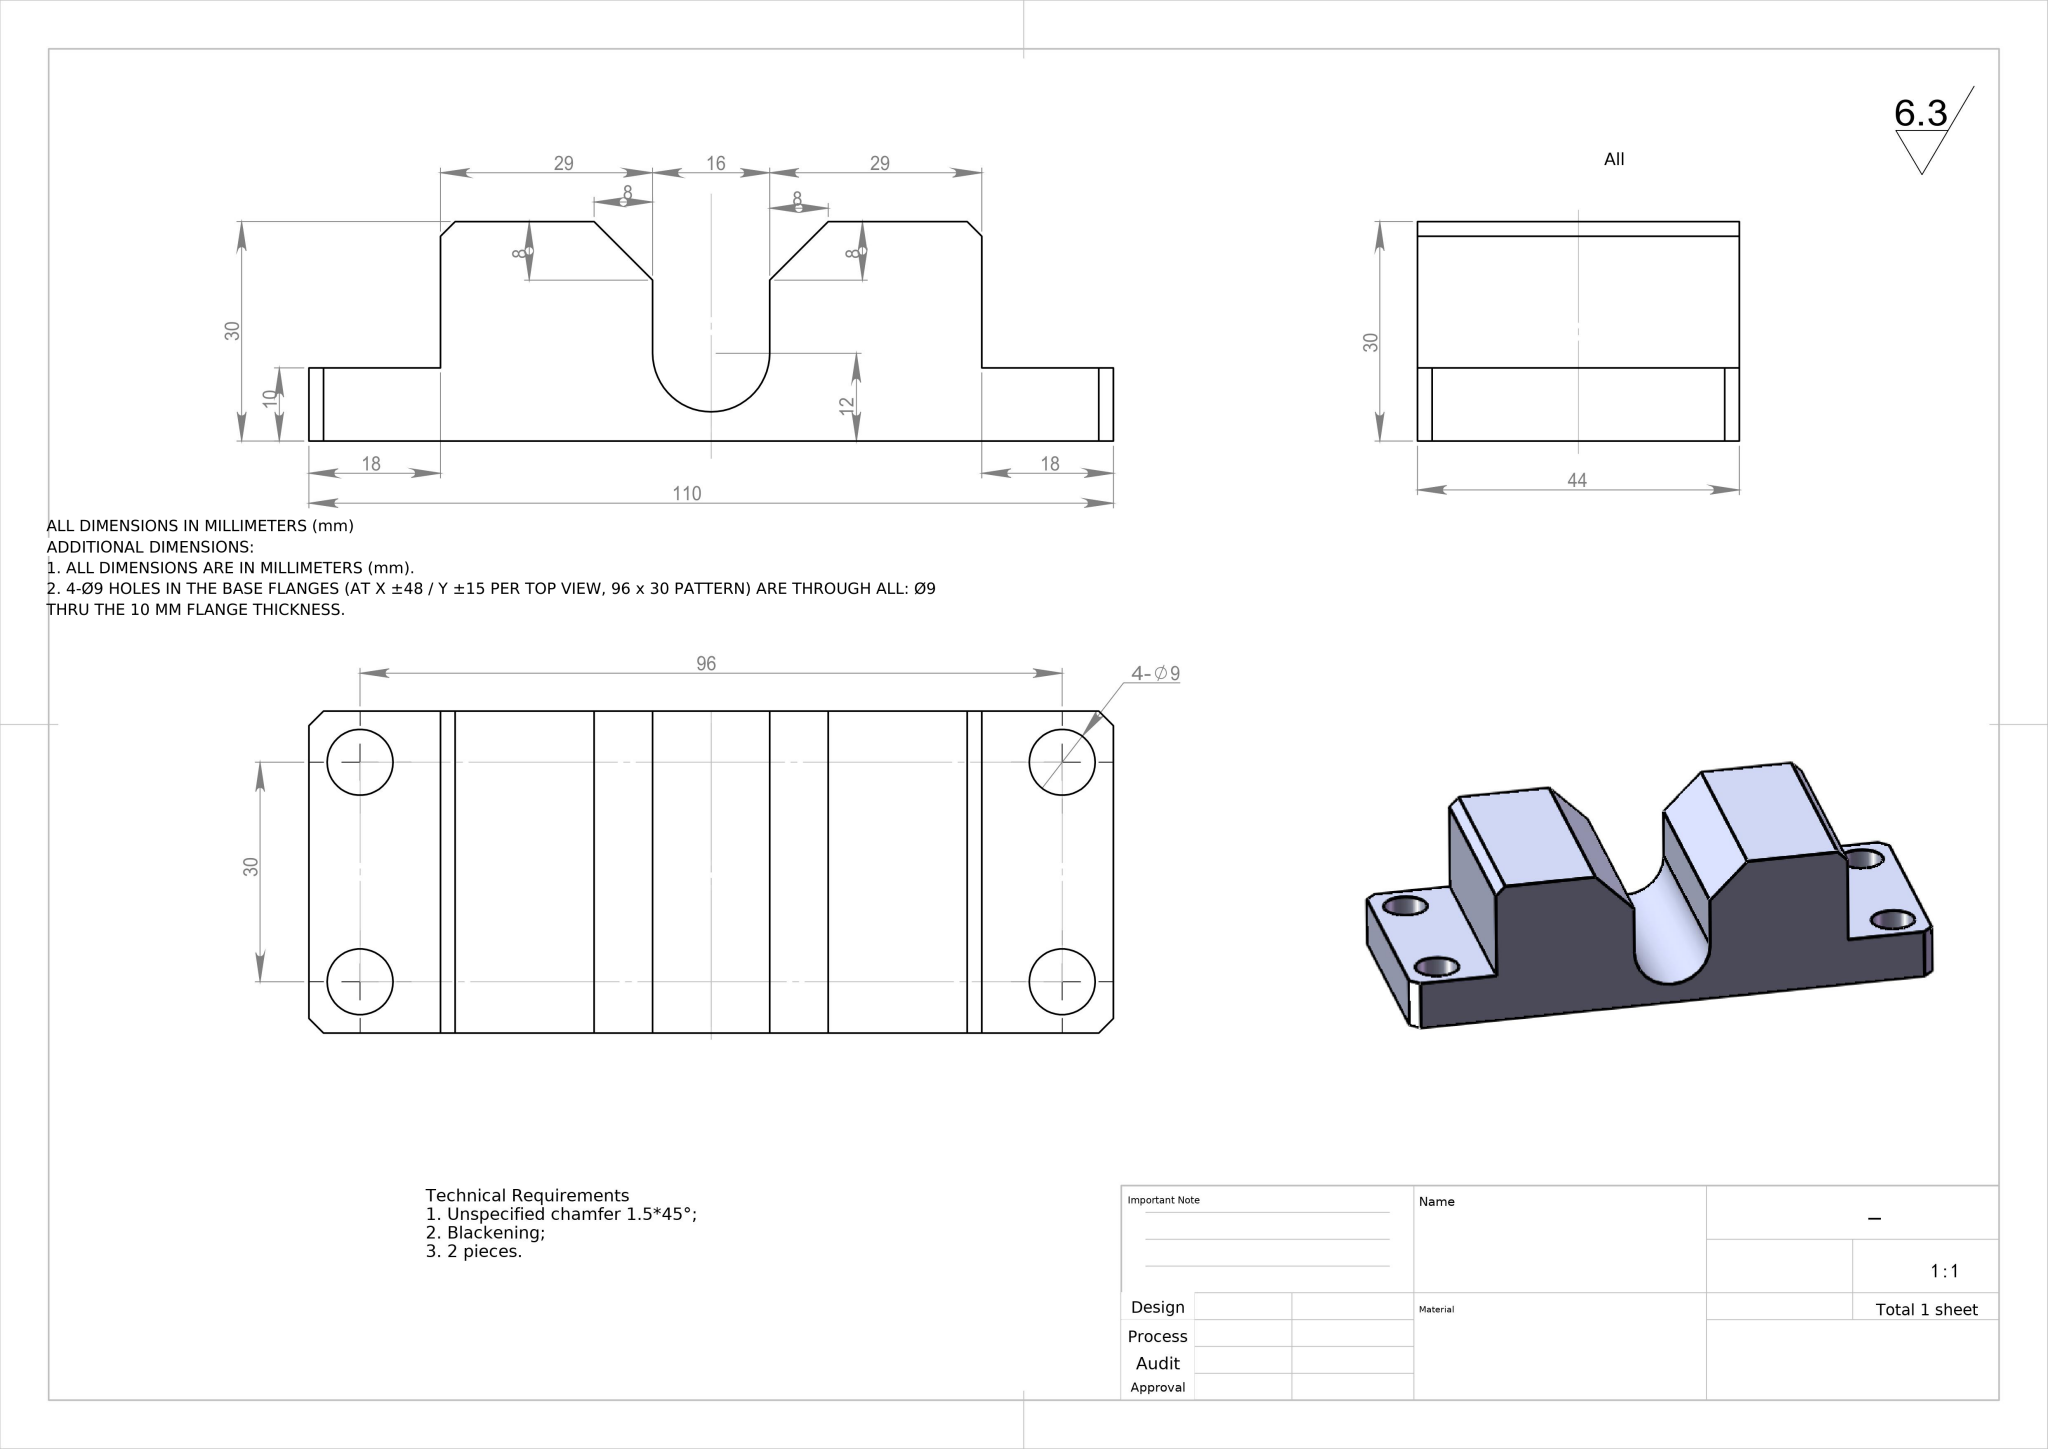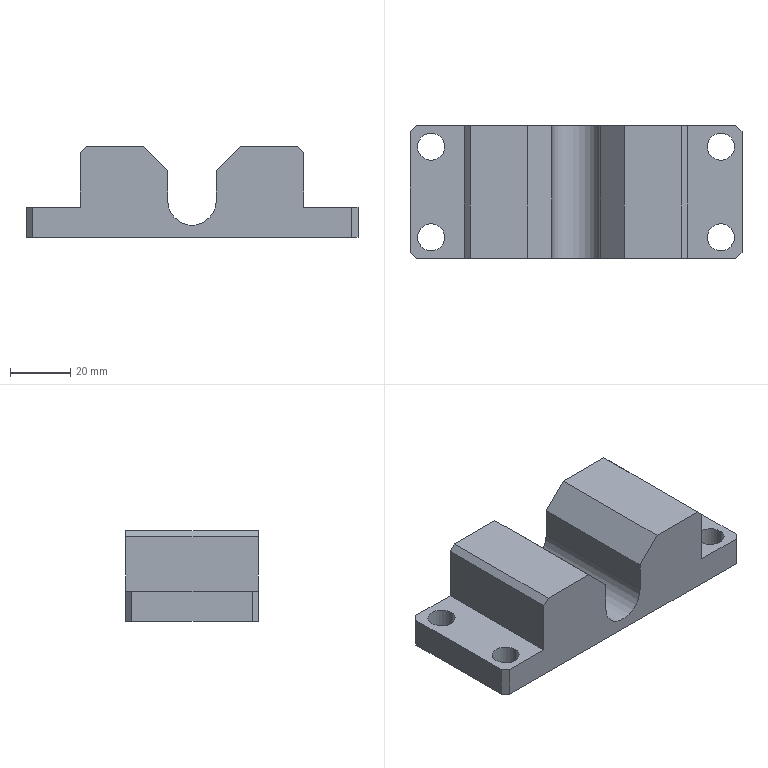Part | NX | mm | Dual-Saddle Tube Mounting Block | 1 solid | 30 faces | box 110 x 44 x 30 mm | volume 90808 mm3 | plane 21 | cylinder 9 | commonest cylinder face diameters 9 x8 16 x1
STEP:
#1=COLOUR_RGB('',0.7961,0.8235,0.9373);
#2=FILL_AREA_STYLE_COLOUR('',#1);
#3=FILL_AREA_STYLE('',(#2));
#4=SURFACE_STYLE_FILL_AREA(#3);
#5=SURFACE_SIDE_STYLE('',(#4));
#6=SURFACE_STYLE_USAGE(.BOTH.,#5);
#7=PRESENTATION_STYLE_ASSIGNMENT((#6));
#8=CARTESIAN_POINT('',(43.5,-15.,0.));
#9=VERTEX_POINT('',#8);
#10=CARTESIAN_POINT('',(52.5,-15.,0.));
#11=VERTEX_POINT('',#10);
#12=CARTESIAN_POINT('',(48.,-15.,0.));
#13=DIRECTION('',(0.,0.,1.));
#14=DIRECTION('',(1.,0.,0.));
#15=AXIS2_PLACEMENT_3D('',#12,#13,#14);
#16=CIRCLE('',#15,4.5);
#17=EDGE_CURVE('',#9,#11,#16,.T.);
#18=ORIENTED_EDGE('',*,*,#17,.F.);
#19=CARTESIAN_POINT('',(43.5,-15.,10.));
#20=VERTEX_POINT('',#19);
#21=CARTESIAN_POINT('',(43.5,-15.,0.));
#22=DIRECTION('',(0.,0.,1.));
#23=VECTOR('',#22,1000.);
#24=LINE('',#21,#23);
#25=EDGE_CURVE('',#9,#20,#24,.T.);
#26=ORIENTED_EDGE('',*,*,#25,.T.);
#27=CARTESIAN_POINT('',(52.5,-15.,10.));
#28=VERTEX_POINT('',#27);
#29=CARTESIAN_POINT('',(48.,-15.,10.));
#30=DIRECTION('',(0.,0.,1.));
#31=DIRECTION('',(-1.,0.,0.));
#32=AXIS2_PLACEMENT_3D('',#29,#30,#31);
#33=CIRCLE('',#32,4.5);
#34=EDGE_CURVE('',#20,#28,#33,.T.);
#35=ORIENTED_EDGE('',*,*,#34,.T.);
#36=CARTESIAN_POINT('',(52.5,-15.,0.));
#37=DIRECTION('',(0.,0.,1.));
#38=VECTOR('',#37,1000.);
#39=LINE('',#36,#38);
#40=EDGE_CURVE('',#11,#28,#39,.T.);
#41=ORIENTED_EDGE('',*,*,#40,.F.);
#42=EDGE_LOOP('',(#18,#26,#35,#41));
#43=FACE_OUTER_BOUND('',#42,.T.);
#44=CARTESIAN_POINT('',(48.,-15.,0.));
#45=DIRECTION('',(0.,0.,1.));
#46=DIRECTION('',(1.,0.,0.));
#47=AXIS2_PLACEMENT_3D('',#44,#45,#46);
#48=CYLINDRICAL_SURFACE('',#47,4.5);
#49=ADVANCED_FACE('',(#43),#48,.F.);
#50=CARTESIAN_POINT('',(43.5,15.,0.));
#51=VERTEX_POINT('',#50);
#52=CARTESIAN_POINT('',(52.5,15.,0.));
#53=VERTEX_POINT('',#52);
#54=CARTESIAN_POINT('',(48.,15.,0.));
#55=DIRECTION('',(0.,0.,1.));
#56=DIRECTION('',(1.,0.,0.));
#57=AXIS2_PLACEMENT_3D('',#54,#55,#56);
#58=CIRCLE('',#57,4.5);
#59=EDGE_CURVE('',#51,#53,#58,.T.);
#60=ORIENTED_EDGE('',*,*,#59,.F.);
#61=CARTESIAN_POINT('',(43.5,15.,10.));
#62=VERTEX_POINT('',#61);
#63=CARTESIAN_POINT('',(43.5,15.,0.));
#64=DIRECTION('',(0.,0.,1.));
#65=VECTOR('',#64,1000.);
#66=LINE('',#63,#65);
#67=EDGE_CURVE('',#51,#62,#66,.T.);
#68=ORIENTED_EDGE('',*,*,#67,.T.);
#69=CARTESIAN_POINT('',(52.5,15.,10.));
#70=VERTEX_POINT('',#69);
#71=CARTESIAN_POINT('',(48.,15.,10.));
#72=DIRECTION('',(0.,0.,1.));
#73=DIRECTION('',(-1.,0.,0.));
#74=AXIS2_PLACEMENT_3D('',#71,#72,#73);
#75=CIRCLE('',#74,4.5);
#76=EDGE_CURVE('',#62,#70,#75,.T.);
#77=ORIENTED_EDGE('',*,*,#76,.T.);
#78=CARTESIAN_POINT('',(52.5,15.,0.));
#79=DIRECTION('',(0.,0.,1.));
#80=VECTOR('',#79,1000.);
#81=LINE('',#78,#80);
#82=EDGE_CURVE('',#53,#70,#81,.T.);
#83=ORIENTED_EDGE('',*,*,#82,.F.);
#84=EDGE_LOOP('',(#60,#68,#77,#83));
#85=FACE_OUTER_BOUND('',#84,.T.);
#86=CARTESIAN_POINT('',(48.,15.,0.));
#87=DIRECTION('',(0.,0.,1.));
#88=DIRECTION('',(1.,0.,0.));
#89=AXIS2_PLACEMENT_3D('',#86,#87,#88);
#90=CYLINDRICAL_SURFACE('',#89,4.5);
#91=ADVANCED_FACE('',(#85),#90,.F.);
#92=CARTESIAN_POINT('',(-52.5,15.,0.));
#93=VERTEX_POINT('',#92);
#94=CARTESIAN_POINT('',(-43.5,15.,0.));
#95=VERTEX_POINT('',#94);
#96=CARTESIAN_POINT('',(-48.,15.,0.));
#97=DIRECTION('',(0.,0.,1.));
#98=DIRECTION('',(1.,0.,0.));
#99=AXIS2_PLACEMENT_3D('',#96,#97,#98);
#100=CIRCLE('',#99,4.5);
#101=EDGE_CURVE('',#93,#95,#100,.T.);
#102=ORIENTED_EDGE('',*,*,#101,.F.);
#103=CARTESIAN_POINT('',(-52.5,15.,10.));
#104=VERTEX_POINT('',#103);
#105=CARTESIAN_POINT('',(-52.5,15.,0.));
#106=DIRECTION('',(0.,0.,1.));
#107=VECTOR('',#106,1000.);
#108=LINE('',#105,#107);
#109=EDGE_CURVE('',#93,#104,#108,.T.);
#110=ORIENTED_EDGE('',*,*,#109,.T.);
#111=CARTESIAN_POINT('',(-43.5,15.,10.));
#112=VERTEX_POINT('',#111);
#113=CARTESIAN_POINT('',(-48.,15.,10.));
#114=DIRECTION('',(0.,0.,-1.));
#115=DIRECTION('',(1.,0.,0.));
#116=AXIS2_PLACEMENT_3D('',#113,#114,#115);
#117=CIRCLE('',#116,4.5);
#118=EDGE_CURVE('',#112,#104,#117,.T.);
#119=ORIENTED_EDGE('',*,*,#118,.F.);
#120=CARTESIAN_POINT('',(-43.5,15.,0.));
#121=DIRECTION('',(0.,0.,1.));
#122=VECTOR('',#121,1000.);
#123=LINE('',#120,#122);
#124=EDGE_CURVE('',#95,#112,#123,.T.);
#125=ORIENTED_EDGE('',*,*,#124,.F.);
#126=EDGE_LOOP('',(#102,#110,#119,#125));
#127=FACE_OUTER_BOUND('',#126,.T.);
#128=CARTESIAN_POINT('',(-48.,15.,0.));
#129=DIRECTION('',(0.,0.,1.));
#130=DIRECTION('',(1.,0.,0.));
#131=AXIS2_PLACEMENT_3D('',#128,#129,#130);
#132=CYLINDRICAL_SURFACE('',#131,4.5);
#133=ADVANCED_FACE('',(#127),#132,.F.);
#134=CARTESIAN_POINT('',(-52.5,-15.,0.));
#135=VERTEX_POINT('',#134);
#136=CARTESIAN_POINT('',(-43.5,-15.,0.));
#137=VERTEX_POINT('',#136);
#138=CARTESIAN_POINT('',(-48.,-15.,0.));
#139=DIRECTION('',(0.,0.,1.));
#140=DIRECTION('',(1.,0.,0.));
#141=AXIS2_PLACEMENT_3D('',#138,#139,#140);
#142=CIRCLE('',#141,4.5);
#143=EDGE_CURVE('',#135,#137,#142,.T.);
#144=ORIENTED_EDGE('',*,*,#143,.F.);
#145=CARTESIAN_POINT('',(-52.5,-15.,10.));
#146=VERTEX_POINT('',#145);
#147=CARTESIAN_POINT('',(-52.5,-15.,0.));
#148=DIRECTION('',(0.,0.,1.));
#149=VECTOR('',#148,1000.);
#150=LINE('',#147,#149);
#151=EDGE_CURVE('',#135,#146,#150,.T.);
#152=ORIENTED_EDGE('',*,*,#151,.T.);
#153=CARTESIAN_POINT('',(-43.5,-15.,10.));
#154=VERTEX_POINT('',#153);
#155=CARTESIAN_POINT('',(-48.,-15.,10.));
#156=DIRECTION('',(0.,0.,-1.));
#157=DIRECTION('',(1.,0.,0.));
#158=AXIS2_PLACEMENT_3D('',#155,#156,#157);
#159=CIRCLE('',#158,4.5);
#160=EDGE_CURVE('',#154,#146,#159,.T.);
#161=ORIENTED_EDGE('',*,*,#160,.F.);
#162=CARTESIAN_POINT('',(-43.5,-15.,0.));
#163=DIRECTION('',(0.,0.,1.));
#164=VECTOR('',#163,1000.);
#165=LINE('',#162,#164);
#166=EDGE_CURVE('',#137,#154,#165,.T.);
#167=ORIENTED_EDGE('',*,*,#166,.F.);
#168=EDGE_LOOP('',(#144,#152,#161,#167));
#169=FACE_OUTER_BOUND('',#168,.T.);
#170=CARTESIAN_POINT('',(-48.,-15.,0.));
#171=DIRECTION('',(0.,0.,1.));
#172=DIRECTION('',(1.,0.,0.));
#173=AXIS2_PLACEMENT_3D('',#170,#171,#172);
#174=CYLINDRICAL_SURFACE('',#173,4.5);
#175=ADVANCED_FACE('',(#169),#174,.F.);
#176=CARTESIAN_POINT('',(-55.,20.,10.));
#177=VERTEX_POINT('',#176);
#178=CARTESIAN_POINT('',(-55.,-20.,10.));
#179=VERTEX_POINT('',#178);
#180=CARTESIAN_POINT('',(-55.,22.,10.));
#181=DIRECTION('',(0.,-1.,0.));
#182=VECTOR('',#181,1000.);
#183=LINE('',#180,#182);
#184=EDGE_CURVE('',#177,#179,#183,.T.);
#185=ORIENTED_EDGE('',*,*,#184,.F.);
#186=CARTESIAN_POINT('',(-55.,20.,0.));
#187=VERTEX_POINT('',#186);
#188=CARTESIAN_POINT('',(-55.,20.,30.));
#189=DIRECTION('',(0.,0.,-1.));
#190=VECTOR('',#189,1000.);
#191=LINE('',#188,#190);
#192=EDGE_CURVE('',#177,#187,#191,.T.);
#193=ORIENTED_EDGE('',*,*,#192,.T.);
#194=CARTESIAN_POINT('',(-55.,-20.,0.));
#195=VERTEX_POINT('',#194);
#196=CARTESIAN_POINT('',(-55.,22.,0.));
#197=DIRECTION('',(-0.,-1.,0.));
#198=VECTOR('',#197,1000.);
#199=LINE('',#196,#198);
#200=EDGE_CURVE('',#187,#195,#199,.T.);
#201=ORIENTED_EDGE('',*,*,#200,.T.);
#202=CARTESIAN_POINT('',(-55.,-20.,30.));
#203=DIRECTION('',(0.,0.,1.));
#204=VECTOR('',#203,1000.);
#205=LINE('',#202,#204);
#206=EDGE_CURVE('',#195,#179,#205,.T.);
#207=ORIENTED_EDGE('',*,*,#206,.T.);
#208=EDGE_LOOP('',(#185,#193,#201,#207));
#209=FACE_OUTER_BOUND('',#208,.T.);
#210=CARTESIAN_POINT('',(-55.,22.,30.));
#211=DIRECTION('',(1.,-0.,0.));
#212=DIRECTION('',(0.,1.,0.));
#213=AXIS2_PLACEMENT_3D('',#210,#211,#212);
#214=PLANE('',#213);
#215=ADVANCED_FACE('',(#209),#214,.F.);
#216=ORIENTED_EDGE('',*,*,#151,.F.);
#217=CARTESIAN_POINT('',(-48.,-15.,0.));
#218=DIRECTION('',(0.,0.,1.));
#219=DIRECTION('',(1.,0.,0.));
#220=AXIS2_PLACEMENT_3D('',#217,#218,#219);
#221=CIRCLE('',#220,4.5);
#222=EDGE_CURVE('',#137,#135,#221,.T.);
#223=ORIENTED_EDGE('',*,*,#222,.F.);
#224=ORIENTED_EDGE('',*,*,#166,.T.);
#225=CARTESIAN_POINT('',(-48.,-15.,10.));
#226=DIRECTION('',(0.,0.,-1.));
#227=DIRECTION('',(1.,0.,0.));
#228=AXIS2_PLACEMENT_3D('',#225,#226,#227);
#229=CIRCLE('',#228,4.5);
#230=EDGE_CURVE('',#146,#154,#229,.T.);
#231=ORIENTED_EDGE('',*,*,#230,.F.);
#232=EDGE_LOOP('',(#216,#223,#224,#231));
#233=FACE_OUTER_BOUND('',#232,.T.);
#234=CARTESIAN_POINT('',(-48.,-15.,0.));
#235=DIRECTION('',(0.,0.,1.));
#236=DIRECTION('',(1.,0.,0.));
#237=AXIS2_PLACEMENT_3D('',#234,#235,#236);
#238=CYLINDRICAL_SURFACE('',#237,4.5);
#239=ADVANCED_FACE('',(#233),#238,.F.);
#240=ORIENTED_EDGE('',*,*,#109,.F.);
#241=CARTESIAN_POINT('',(-48.,15.,0.));
#242=DIRECTION('',(0.,0.,1.));
#243=DIRECTION('',(1.,0.,0.));
#244=AXIS2_PLACEMENT_3D('',#241,#242,#243);
#245=CIRCLE('',#244,4.5);
#246=EDGE_CURVE('',#95,#93,#245,.T.);
#247=ORIENTED_EDGE('',*,*,#246,.F.);
#248=ORIENTED_EDGE('',*,*,#124,.T.);
#249=CARTESIAN_POINT('',(-48.,15.,10.));
#250=DIRECTION('',(0.,0.,-1.));
#251=DIRECTION('',(1.,0.,0.));
#252=AXIS2_PLACEMENT_3D('',#249,#250,#251);
#253=CIRCLE('',#252,4.5);
#254=EDGE_CURVE('',#104,#112,#253,.T.);
#255=ORIENTED_EDGE('',*,*,#254,.F.);
#256=EDGE_LOOP('',(#240,#247,#248,#255));
#257=FACE_OUTER_BOUND('',#256,.T.);
#258=CARTESIAN_POINT('',(-48.,15.,0.));
#259=DIRECTION('',(0.,0.,1.));
#260=DIRECTION('',(1.,0.,0.));
#261=AXIS2_PLACEMENT_3D('',#258,#259,#260);
#262=CYLINDRICAL_SURFACE('',#261,4.5);
#263=ADVANCED_FACE('',(#257),#262,.F.);
#264=CARTESIAN_POINT('',(35.,22.,30.));
#265=VERTEX_POINT('',#264);
#266=CARTESIAN_POINT('',(16.,22.,30.));
#267=VERTEX_POINT('',#266);
#268=CARTESIAN_POINT('',(-55.,22.,30.));
#269=DIRECTION('',(-1.,-0.,0.));
#270=VECTOR('',#269,1000.);
#271=LINE('',#268,#270);
#272=EDGE_CURVE('',#265,#267,#271,.T.);
#273=ORIENTED_EDGE('',*,*,#272,.T.);
#274=CARTESIAN_POINT('',(16.,-22.,30.));
#275=VERTEX_POINT('',#274);
#276=CARTESIAN_POINT('',(16.,-22.,30.));
#277=DIRECTION('',(0.,-1.,0.));
#278=VECTOR('',#277,1000.);
#279=LINE('',#276,#278);
#280=EDGE_CURVE('',#267,#275,#279,.T.);
#281=ORIENTED_EDGE('',*,*,#280,.T.);
#282=CARTESIAN_POINT('',(35.,-22.,30.));
#283=VERTEX_POINT('',#282);
#284=CARTESIAN_POINT('',(-55.,-22.,30.));
#285=DIRECTION('',(1.,0.,0.));
#286=VECTOR('',#285,1000.);
#287=LINE('',#284,#286);
#288=EDGE_CURVE('',#275,#283,#287,.T.);
#289=ORIENTED_EDGE('',*,*,#288,.T.);
#290=CARTESIAN_POINT('',(35.,22.,30.));
#291=DIRECTION('',(-0.,1.,0.));
#292=VECTOR('',#291,1000.);
#293=LINE('',#290,#292);
#294=EDGE_CURVE('',#283,#265,#293,.T.);
#295=ORIENTED_EDGE('',*,*,#294,.T.);
#296=EDGE_LOOP('',(#273,#281,#289,#295));
#297=FACE_OUTER_BOUND('',#296,.T.);
#298=CARTESIAN_POINT('',(0.,0.,30.));
#299=DIRECTION('',(0.,0.,1.));
#300=DIRECTION('',(1.,0.,0.));
#301=AXIS2_PLACEMENT_3D('',#298,#299,#300);
#302=PLANE('',#301);
#303=ADVANCED_FACE('',(#297),#302,.T.);
#304=CARTESIAN_POINT('',(55.,-20.,0.));
#305=VERTEX_POINT('',#304);
#306=CARTESIAN_POINT('',(55.,20.,0.));
#307=VERTEX_POINT('',#306);
#308=CARTESIAN_POINT('',(55.,22.,0.));
#309=DIRECTION('',(0.,1.,0.));
#310=VECTOR('',#309,1000.);
#311=LINE('',#308,#310);
#312=EDGE_CURVE('',#305,#307,#311,.T.);
#313=ORIENTED_EDGE('',*,*,#312,.T.);
#314=CARTESIAN_POINT('',(55.,20.,10.));
#315=VERTEX_POINT('',#314);
#316=CARTESIAN_POINT('',(55.,20.,30.));
#317=DIRECTION('',(0.,0.,1.));
#318=VECTOR('',#317,1000.);
#319=LINE('',#316,#318);
#320=EDGE_CURVE('',#307,#315,#319,.T.);
#321=ORIENTED_EDGE('',*,*,#320,.T.);
#322=CARTESIAN_POINT('',(55.,-20.,10.));
#323=VERTEX_POINT('',#322);
#324=CARTESIAN_POINT('',(55.,22.,10.));
#325=DIRECTION('',(-0.,1.,0.));
#326=VECTOR('',#325,1000.);
#327=LINE('',#324,#326);
#328=EDGE_CURVE('',#323,#315,#327,.T.);
#329=ORIENTED_EDGE('',*,*,#328,.F.);
#330=CARTESIAN_POINT('',(55.,-20.,30.));
#331=DIRECTION('',(0.,0.,-1.));
#332=VECTOR('',#331,1000.);
#333=LINE('',#330,#332);
#334=EDGE_CURVE('',#323,#305,#333,.T.);
#335=ORIENTED_EDGE('',*,*,#334,.T.);
#336=EDGE_LOOP('',(#313,#321,#329,#335));
#337=FACE_OUTER_BOUND('',#336,.T.);
#338=CARTESIAN_POINT('',(55.,22.,30.));
#339=DIRECTION('',(-1.,0.,0.));
#340=DIRECTION('',(0.,0.,1.));
#341=AXIS2_PLACEMENT_3D('',#338,#339,#340);
#342=PLANE('',#341);
#343=ADVANCED_FACE('',(#337),#342,.F.);
#344=CARTESIAN_POINT('',(-16.,22.,30.));
#345=VERTEX_POINT('',#344);
#346=CARTESIAN_POINT('',(-35.,22.,30.));
#347=VERTEX_POINT('',#346);
#348=CARTESIAN_POINT('',(-55.,22.,30.));
#349=DIRECTION('',(-1.,-0.,0.));
#350=VECTOR('',#349,1000.);
#351=LINE('',#348,#350);
#352=EDGE_CURVE('',#345,#347,#351,.T.);
#353=ORIENTED_EDGE('',*,*,#352,.F.);
#354=CARTESIAN_POINT('',(-8.,22.,22.));
#355=VERTEX_POINT('',#354);
#356=CARTESIAN_POINT('',(-16.,22.,30.));
#357=DIRECTION('',(0.7071,0.,-0.7071));
#358=VECTOR('',#357,1000.);
#359=LINE('',#356,#358);
#360=EDGE_CURVE('',#345,#355,#359,.T.);
#361=ORIENTED_EDGE('',*,*,#360,.T.);
#362=CARTESIAN_POINT('',(-8.,22.,12.));
#363=VERTEX_POINT('',#362);
#364=CARTESIAN_POINT('',(-8.,22.,30.));
#365=DIRECTION('',(0.,0.,1.));
#366=VECTOR('',#365,1000.);
#367=LINE('',#364,#366);
#368=EDGE_CURVE('',#363,#355,#367,.T.);
#369=ORIENTED_EDGE('',*,*,#368,.F.);
#370=CARTESIAN_POINT('',(8.,22.,12.));
#371=VERTEX_POINT('',#370);
#372=CARTESIAN_POINT('',(-0.,22.,12.));
#373=DIRECTION('',(-0.,1.,0.));
#374=DIRECTION('',(-1.,-0.,0.));
#375=AXIS2_PLACEMENT_3D('',#372,#373,#374);
#376=CIRCLE('',#375,8.);
#377=EDGE_CURVE('',#371,#363,#376,.T.);
#378=ORIENTED_EDGE('',*,*,#377,.F.);
#379=CARTESIAN_POINT('',(8.,22.,22.));
#380=VERTEX_POINT('',#379);
#381=CARTESIAN_POINT('',(8.,22.,30.));
#382=DIRECTION('',(0.,0.,-1.));
#383=VECTOR('',#382,1000.);
#384=LINE('',#381,#383);
#385=EDGE_CURVE('',#380,#371,#384,.T.);
#386=ORIENTED_EDGE('',*,*,#385,.F.);
#387=CARTESIAN_POINT('',(8.,22.,22.));
#388=DIRECTION('',(0.7071,0.,0.7071));
#389=VECTOR('',#388,1000.);
#390=LINE('',#387,#389);
#391=EDGE_CURVE('',#380,#267,#390,.T.);
#392=ORIENTED_EDGE('',*,*,#391,.T.);
#393=ORIENTED_EDGE('',*,*,#272,.F.);
#394=CARTESIAN_POINT('',(37.,22.,28.));
#395=VERTEX_POINT('',#394);
#396=CARTESIAN_POINT('',(37.,22.,28.));
#397=DIRECTION('',(0.7071,0.,-0.7071));
#398=VECTOR('',#397,1000.);
#399=LINE('',#396,#398);
#400=EDGE_CURVE('',#265,#395,#399,.T.);
#401=ORIENTED_EDGE('',*,*,#400,.T.);
#402=CARTESIAN_POINT('',(37.,22.,10.));
#403=VERTEX_POINT('',#402);
#404=CARTESIAN_POINT('',(37.,22.,10.));
#405=DIRECTION('',(0.,0.,1.));
#406=VECTOR('',#405,1000.);
#407=LINE('',#404,#406);
#408=EDGE_CURVE('',#403,#395,#407,.T.);
#409=ORIENTED_EDGE('',*,*,#408,.F.);
#410=CARTESIAN_POINT('',(53.,22.,10.));
#411=VERTEX_POINT('',#410);
#412=CARTESIAN_POINT('',(55.,22.,10.));
#413=DIRECTION('',(-1.,-0.,0.));
#414=VECTOR('',#413,1000.);
#415=LINE('',#412,#414);
#416=EDGE_CURVE('',#411,#403,#415,.T.);
#417=ORIENTED_EDGE('',*,*,#416,.F.);
#418=CARTESIAN_POINT('',(53.,22.,0.));
#419=VERTEX_POINT('',#418);
#420=CARTESIAN_POINT('',(53.,22.,30.));
#421=DIRECTION('',(0.,0.,-1.));
#422=VECTOR('',#421,1000.);
#423=LINE('',#420,#422);
#424=EDGE_CURVE('',#411,#419,#423,.T.);
#425=ORIENTED_EDGE('',*,*,#424,.T.);
#426=CARTESIAN_POINT('',(-53.,22.,0.));
#427=VERTEX_POINT('',#426);
#428=CARTESIAN_POINT('',(-55.,22.,0.));
#429=DIRECTION('',(-1.,-0.,0.));
#430=VECTOR('',#429,1000.);
#431=LINE('',#428,#430);
#432=EDGE_CURVE('',#419,#427,#431,.T.);
#433=ORIENTED_EDGE('',*,*,#432,.T.);
#434=CARTESIAN_POINT('',(-53.,22.,10.));
#435=VERTEX_POINT('',#434);
#436=CARTESIAN_POINT('',(-53.,22.,30.));
#437=DIRECTION('',(0.,0.,1.));
#438=VECTOR('',#437,1000.);
#439=LINE('',#436,#438);
#440=EDGE_CURVE('',#427,#435,#439,.T.);
#441=ORIENTED_EDGE('',*,*,#440,.T.);
#442=CARTESIAN_POINT('',(-37.,22.,10.));
#443=VERTEX_POINT('',#442);
#444=CARTESIAN_POINT('',(-55.,22.,10.));
#445=DIRECTION('',(-1.,0.,0.));
#446=VECTOR('',#445,1000.);
#447=LINE('',#444,#446);
#448=EDGE_CURVE('',#443,#435,#447,.T.);
#449=ORIENTED_EDGE('',*,*,#448,.F.);
#450=CARTESIAN_POINT('',(-37.,22.,28.));
#451=VERTEX_POINT('',#450);
#452=CARTESIAN_POINT('',(-37.,22.,10.));
#453=DIRECTION('',(0.,0.,1.));
#454=VECTOR('',#453,1000.);
#455=LINE('',#452,#454);
#456=EDGE_CURVE('',#443,#451,#455,.T.);
#457=ORIENTED_EDGE('',*,*,#456,.T.);
#458=CARTESIAN_POINT('',(-37.,22.,28.));
#459=DIRECTION('',(0.7071,0.,0.7071));
#460=VECTOR('',#459,1000.);
#461=LINE('',#458,#460);
#462=EDGE_CURVE('',#451,#347,#461,.T.);
#463=ORIENTED_EDGE('',*,*,#462,.T.);
#464=EDGE_LOOP('',(#353,#361,#369,#378,#386,#392,#393,#401,#409,#417,#425,#433,#441,#449,#457,#463));
#465=FACE_OUTER_BOUND('',#464,.T.);
#466=CARTESIAN_POINT('',(-55.,22.,30.));
#467=DIRECTION('',(0.,-1.,0.));
#468=DIRECTION('',(1.,0.,0.));
#469=AXIS2_PLACEMENT_3D('',#466,#467,#468);
#470=PLANE('',#469);
#471=ADVANCED_FACE('',(#465),#470,.F.);
#472=CARTESIAN_POINT('',(-8.,-22.,12.));
#473=VERTEX_POINT('',#472);
#474=CARTESIAN_POINT('',(-8.,-22.,22.));
#475=VERTEX_POINT('',#474);
#476=CARTESIAN_POINT('',(-8.,-22.,30.));
#477=DIRECTION('',(0.,0.,1.));
#478=VECTOR('',#477,1000.);
#479=LINE('',#476,#478);
#480=EDGE_CURVE('',#473,#475,#479,.T.);
#481=ORIENTED_EDGE('',*,*,#480,.T.);
#482=CARTESIAN_POINT('',(-16.,-22.,30.));
#483=VERTEX_POINT('',#482);
#484=CARTESIAN_POINT('',(-16.,-22.,30.));
#485=DIRECTION('',(-0.7071,-0.,0.7071));
#486=VECTOR('',#485,1000.);
#487=LINE('',#484,#486);
#488=EDGE_CURVE('',#475,#483,#487,.T.);
#489=ORIENTED_EDGE('',*,*,#488,.T.);
#490=CARTESIAN_POINT('',(-35.,-22.,30.));
#491=VERTEX_POINT('',#490);
#492=CARTESIAN_POINT('',(-55.,-22.,30.));
#493=DIRECTION('',(1.,0.,0.));
#494=VECTOR('',#493,1000.);
#495=LINE('',#492,#494);
#496=EDGE_CURVE('',#491,#483,#495,.T.);
#497=ORIENTED_EDGE('',*,*,#496,.F.);
#498=CARTESIAN_POINT('',(-37.,-22.,28.));
#499=VERTEX_POINT('',#498);
#500=CARTESIAN_POINT('',(-37.,-22.,28.));
#501=DIRECTION('',(-0.7071,-0.,-0.7071));
#502=VECTOR('',#501,1000.);
#503=LINE('',#500,#502);
#504=EDGE_CURVE('',#491,#499,#503,.T.);
#505=ORIENTED_EDGE('',*,*,#504,.T.);
#506=CARTESIAN_POINT('',(-37.,-22.,10.));
#507=VERTEX_POINT('',#506);
#508=CARTESIAN_POINT('',(-37.,-22.,10.));
#509=DIRECTION('',(0.,0.,1.));
#510=VECTOR('',#509,1000.);
#511=LINE('',#508,#510);
#512=EDGE_CURVE('',#507,#499,#511,.T.);
#513=ORIENTED_EDGE('',*,*,#512,.F.);
#514=CARTESIAN_POINT('',(-53.,-22.,10.));
#515=VERTEX_POINT('',#514);
#516=CARTESIAN_POINT('',(-55.,-22.,10.));
#517=DIRECTION('',(1.,0.,0.));
#518=VECTOR('',#517,1000.);
#519=LINE('',#516,#518);
#520=EDGE_CURVE('',#515,#507,#519,.T.);
#521=ORIENTED_EDGE('',*,*,#520,.F.);
#522=CARTESIAN_POINT('',(-53.,-22.,0.));
#523=VERTEX_POINT('',#522);
#524=CARTESIAN_POINT('',(-53.,-22.,30.));
#525=DIRECTION('',(0.,0.,-1.));
#526=VECTOR('',#525,1000.);
#527=LINE('',#524,#526);
#528=EDGE_CURVE('',#515,#523,#527,.T.);
#529=ORIENTED_EDGE('',*,*,#528,.T.);
#530=CARTESIAN_POINT('',(53.,-22.,0.));
#531=VERTEX_POINT('',#530);
#532=CARTESIAN_POINT('',(-55.,-22.,0.));
#533=DIRECTION('',(1.,0.,0.));
#534=VECTOR('',#533,1000.);
#535=LINE('',#532,#534);
#536=EDGE_CURVE('',#523,#531,#535,.T.);
#537=ORIENTED_EDGE('',*,*,#536,.T.);
#538=CARTESIAN_POINT('',(53.,-22.,10.));
#539=VERTEX_POINT('',#538);
#540=CARTESIAN_POINT('',(53.,-22.,30.));
#541=DIRECTION('',(0.,0.,1.));
#542=VECTOR('',#541,1000.);
#543=LINE('',#540,#542);
#544=EDGE_CURVE('',#531,#539,#543,.T.);
#545=ORIENTED_EDGE('',*,*,#544,.T.);
#546=CARTESIAN_POINT('',(37.,-22.,10.));
#547=VERTEX_POINT('',#546);
#548=CARTESIAN_POINT('',(55.,-22.,10.));
#549=DIRECTION('',(1.,0.,0.));
#550=VECTOR('',#549,1000.);
#551=LINE('',#548,#550);
#552=EDGE_CURVE('',#547,#539,#551,.T.);
#553=ORIENTED_EDGE('',*,*,#552,.F.);
#554=CARTESIAN_POINT('',(37.,-22.,28.));
#555=VERTEX_POINT('',#554);
#556=CARTESIAN_POINT('',(37.,-22.,10.));
#557=DIRECTION('',(0.,0.,1.));
#558=VECTOR('',#557,1000.);
#559=LINE('',#556,#558);
#560=EDGE_CURVE('',#547,#555,#559,.T.);
#561=ORIENTED_EDGE('',*,*,#560,.T.);
#562=CARTESIAN_POINT('',(37.,-22.,28.));
#563=DIRECTION('',(-0.7071,-0.,0.7071));
#564=VECTOR('',#563,1000.);
#565=LINE('',#562,#564);
#566=EDGE_CURVE('',#555,#283,#565,.T.);
#567=ORIENTED_EDGE('',*,*,#566,.T.);
#568=ORIENTED_EDGE('',*,*,#288,.F.);
#569=CARTESIAN_POINT('',(8.,-22.,22.));
#570=VERTEX_POINT('',#569);
#571=CARTESIAN_POINT('',(8.,-22.,22.));
#572=DIRECTION('',(-0.7071,-0.,-0.7071));
#573=VECTOR('',#572,1000.);
#574=LINE('',#571,#573);
#575=EDGE_CURVE('',#275,#570,#574,.T.);
#576=ORIENTED_EDGE('',*,*,#575,.T.);
#577=CARTESIAN_POINT('',(8.,-22.,12.));
#578=VERTEX_POINT('',#577);
#579=CARTESIAN_POINT('',(8.,-22.,30.));
#580=DIRECTION('',(0.,0.,-1.));
#581=VECTOR('',#580,1000.);
#582=LINE('',#579,#581);
#583=EDGE_CURVE('',#570,#578,#582,.T.);
#584=ORIENTED_EDGE('',*,*,#583,.T.);
#585=CARTESIAN_POINT('',(0.,-22.,12.));
#586=DIRECTION('',(-0.,1.,0.));
#587=DIRECTION('',(-1.,-0.,0.));
#588=AXIS2_PLACEMENT_3D('',#585,#586,#587);
#589=CIRCLE('',#588,8.);
#590=EDGE_CURVE('',#578,#473,#589,.T.);
#591=ORIENTED_EDGE('',*,*,#590,.T.);
#592=EDGE_LOOP('',(#481,#489,#497,#505,#513,#521,#529,#537,#545,#553,#561,#567,#568,#576,#584,#591));
#593=FACE_OUTER_BOUND('',#592,.T.);
#594=CARTESIAN_POINT('',(-55.,-22.,30.));
#595=DIRECTION('',(-0.,1.,0.));
#596=DIRECTION('',(-1.,-0.,0.));
#597=AXIS2_PLACEMENT_3D('',#594,#595,#596);
#598=PLANE('',#597);
#599=ADVANCED_FACE('',(#593),#598,.F.);
#600=ORIENTED_EDGE('',*,*,#496,.T.);
#601=CARTESIAN_POINT('',(-16.,22.,30.));
#602=DIRECTION('',(-0.,1.,0.));
#603=VECTOR('',#602,1000.);
#604=LINE('',#601,#603);
#605=EDGE_CURVE('',#483,#345,#604,.T.);
#606=ORIENTED_EDGE('',*,*,#605,.T.);
#607=ORIENTED_EDGE('',*,*,#352,.T.);
#608=CARTESIAN_POINT('',(-35.,-22.,30.));
#609=DIRECTION('',(0.,-1.,0.));
#610=VECTOR('',#609,1000.);
#611=LINE('',#608,#610);
#612=EDGE_CURVE('',#347,#491,#611,.T.);
#613=ORIENTED_EDGE('',*,*,#612,.T.);
#614=EDGE_LOOP('',(#600,#606,#607,#613));
#615=FACE_OUTER_BOUND('',#614,.T.);
#616=CARTESIAN_POINT('',(0.,0.,30.));
#617=DIRECTION('',(0.,0.,1.));
#618=DIRECTION('',(1.,0.,0.));
#619=AXIS2_PLACEMENT_3D('',#616,#617,#618);
#620=PLANE('',#619);
#621=ADVANCED_FACE('',(#615),#620,.T.);
#622=CARTESIAN_POINT('',(48.,-15.,0.));
#623=DIRECTION('',(0.,0.,1.));
#624=DIRECTION('',(1.,0.,0.));
#625=AXIS2_PLACEMENT_3D('',#622,#623,#624);
#626=CIRCLE('',#625,4.5);
#627=EDGE_CURVE('',#11,#9,#626,.T.);
#628=ORIENTED_EDGE('',*,*,#627,.T.);
#629=ORIENTED_EDGE('',*,*,#17,.T.);
#630=EDGE_LOOP('',(#628,#629));
#631=FACE_BOUND('',#630,.T.);
#632=CARTESIAN_POINT('',(48.,15.,0.));
#633=DIRECTION('',(0.,0.,1.));
#634=DIRECTION('',(1.,0.,0.));
#635=AXIS2_PLACEMENT_3D('',#632,#633,#634);
#636=CIRCLE('',#635,4.5);
#637=EDGE_CURVE('',#53,#51,#636,.T.);
#638=ORIENTED_EDGE('',*,*,#637,.T.);
#639=ORIENTED_EDGE('',*,*,#59,.T.);
#640=EDGE_LOOP('',(#638,#639));
#641=FACE_BOUND('',#640,.T.);
#642=ORIENTED_EDGE('',*,*,#246,.T.);
#643=ORIENTED_EDGE('',*,*,#101,.T.);
#644=EDGE_LOOP('',(#642,#643));
#645=FACE_BOUND('',#644,.T.);
#646=ORIENTED_EDGE('',*,*,#222,.T.);
#647=ORIENTED_EDGE('',*,*,#143,.T.);
#648=EDGE_LOOP('',(#646,#647));
#649=FACE_BOUND('',#648,.T.);
#650=ORIENTED_EDGE('',*,*,#432,.F.);
#651=CARTESIAN_POINT('',(53.,22.,0.));
#652=DIRECTION('',(0.7071,-0.7071,0.));
#653=VECTOR('',#652,1000.);
#654=LINE('',#651,#653);
#655=EDGE_CURVE('',#419,#307,#654,.T.);
#656=ORIENTED_EDGE('',*,*,#655,.T.);
#657=ORIENTED_EDGE('',*,*,#312,.F.);
#658=CARTESIAN_POINT('',(55.,-20.,0.));
#659=DIRECTION('',(-0.7071,-0.7071,0.));
#660=VECTOR('',#659,1000.);
#661=LINE('',#658,#660);
#662=EDGE_CURVE('',#305,#531,#661,.T.);
#663=ORIENTED_EDGE('',*,*,#662,.T.);
#664=ORIENTED_EDGE('',*,*,#536,.F.);
#665=CARTESIAN_POINT('',(-53.,-22.,0.));
#666=DIRECTION('',(-0.7071,0.7071,0.));
#667=VECTOR('',#666,1000.);
#668=LINE('',#665,#667);
#669=EDGE_CURVE('',#523,#195,#668,.T.);
#670=ORIENTED_EDGE('',*,*,#669,.T.);
#671=ORIENTED_EDGE('',*,*,#200,.F.);
#672=CARTESIAN_POINT('',(-55.,20.,0.));
#673=DIRECTION('',(0.7071,0.7071,0.));
#674=VECTOR('',#673,1000.);
#675=LINE('',#672,#674);
#676=EDGE_CURVE('',#187,#427,#675,.T.);
#677=ORIENTED_EDGE('',*,*,#676,.T.);
#678=EDGE_LOOP('',(#650,#656,#657,#663,#664,#670,#671,#677));
#679=FACE_OUTER_BOUND('',#678,.T.);
#680=CARTESIAN_POINT('',(0.,0.,0.));
#681=DIRECTION('',(0.,0.,1.));
#682=DIRECTION('',(1.,0.,0.));
#683=AXIS2_PLACEMENT_3D('',#680,#681,#682);
#684=PLANE('',#683);
#685=ADVANCED_FACE('',(#631,#641,#645,#649,#679),#684,.F.);
#686=ORIENTED_EDGE('',*,*,#377,.T.);
#687=CARTESIAN_POINT('',(-8.,-22.,12.));
#688=DIRECTION('',(-0.,1.,0.));
#689=VECTOR('',#688,1000.);
#690=LINE('',#687,#689);
#691=EDGE_CURVE('',#473,#363,#690,.T.);
#692=ORIENTED_EDGE('',*,*,#691,.F.);
#693=ORIENTED_EDGE('',*,*,#590,.F.);
#694=CARTESIAN_POINT('',(8.,-22.,12.));
#695=DIRECTION('',(-0.,1.,0.));
#696=VECTOR('',#695,1000.);
#697=LINE('',#694,#696);
#698=EDGE_CURVE('',#578,#371,#697,.T.);
#699=ORIENTED_EDGE('',*,*,#698,.T.);
#700=EDGE_LOOP('',(#686,#692,#693,#699));
#701=FACE_OUTER_BOUND('',#700,.T.);
#702=CARTESIAN_POINT('',(0.,-22.,12.));
#703=DIRECTION('',(-0.,1.,0.));
#704=DIRECTION('',(-1.,-0.,0.));
#705=AXIS2_PLACEMENT_3D('',#702,#703,#704);
#706=CYLINDRICAL_SURFACE('',#705,8.);
#707=ADVANCED_FACE('',(#701),#706,.F.);
#708=ORIENTED_EDGE('',*,*,#583,.F.);
#709=CARTESIAN_POINT('',(8.,22.,22.));
#710=DIRECTION('',(-0.,1.,0.));
#711=VECTOR('',#710,1000.);
#712=LINE('',#709,#711);
#713=EDGE_CURVE('',#570,#380,#712,.T.);
#714=ORIENTED_EDGE('',*,*,#713,.T.);
#715=ORIENTED_EDGE('',*,*,#385,.T.);
#716=ORIENTED_EDGE('',*,*,#698,.F.);
#717=EDGE_LOOP('',(#708,#714,#715,#716));
#718=FACE_OUTER_BOUND('',#717,.T.);
#719=CARTESIAN_POINT('',(8.,-22.,30.));
#720=DIRECTION('',(1.,0.,0.));
#721=DIRECTION('',(-0.,1.,0.));
#722=AXIS2_PLACEMENT_3D('',#719,#720,#721);
#723=PLANE('',#722);
#724=ADVANCED_FACE('',(#718),#723,.F.);
#725=ORIENTED_EDGE('',*,*,#368,.T.);
#726=CARTESIAN_POINT('',(-8.,-22.,22.));
#727=DIRECTION('',(0.,-1.,0.));
#728=VECTOR('',#727,1000.);
#729=LINE('',#726,#728);
#730=EDGE_CURVE('',#355,#475,#729,.T.);
#731=ORIENTED_EDGE('',*,*,#730,.T.);
#732=ORIENTED_EDGE('',*,*,#480,.F.);
#733=ORIENTED_EDGE('',*,*,#691,.T.);
#734=EDGE_LOOP('',(#725,#731,#732,#733));
#735=FACE_OUTER_BOUND('',#734,.T.);
#736=CARTESIAN_POINT('',(-8.,-22.,30.));
#737=DIRECTION('',(-1.,-0.,0.));
#738=DIRECTION('',(0.,-1.,0.));
#739=AXIS2_PLACEMENT_3D('',#736,#737,#738);
#740=PLANE('',#739);
#741=ADVANCED_FACE('',(#735),#740,.F.);
#742=ORIENTED_EDGE('',*,*,#67,.F.);
#743=ORIENTED_EDGE('',*,*,#637,.F.);
#744=ORIENTED_EDGE('',*,*,#82,.T.);
#745=CARTESIAN_POINT('',(48.,15.,10.));
#746=DIRECTION('',(0.,0.,1.));
#747=DIRECTION('',(-1.,0.,0.));
#748=AXIS2_PLACEMENT_3D('',#745,#746,#747);
#749=CIRCLE('',#748,4.5);
#750=EDGE_CURVE('',#70,#62,#749,.T.);
#751=ORIENTED_EDGE('',*,*,#750,.T.);
#752=EDGE_LOOP('',(#742,#743,#744,#751));
#753=FACE_OUTER_BOUND('',#752,.T.);
#754=CARTESIAN_POINT('',(48.,15.,0.));
#755=DIRECTION('',(0.,0.,1.));
#756=DIRECTION('',(1.,0.,0.));
#757=AXIS2_PLACEMENT_3D('',#754,#755,#756);
#758=CYLINDRICAL_SURFACE('',#757,4.5);
#759=ADVANCED_FACE('',(#753),#758,.F.);
#760=ORIENTED_EDGE('',*,*,#25,.F.);
#761=ORIENTED_EDGE('',*,*,#627,.F.);
#762=ORIENTED_EDGE('',*,*,#40,.T.);
#763=CARTESIAN_POINT('',(48.,-15.,10.));
#764=DIRECTION('',(0.,0.,1.));
#765=DIRECTION('',(-1.,0.,0.));
#766=AXIS2_PLACEMENT_3D('',#763,#764,#765);
#767=CIRCLE('',#766,4.5);
#768=EDGE_CURVE('',#28,#20,#767,.T.);
#769=ORIENTED_EDGE('',*,*,#768,.T.);
#770=EDGE_LOOP('',(#760,#761,#762,#769));
#771=FACE_OUTER_BOUND('',#770,.T.);
#772=CARTESIAN_POINT('',(48.,-15.,0.));
#773=DIRECTION('',(0.,0.,1.));
#774=DIRECTION('',(1.,0.,0.));
#775=AXIS2_PLACEMENT_3D('',#772,#773,#774);
#776=CYLINDRICAL_SURFACE('',#775,4.5);
#777=ADVANCED_FACE('',(#771),#776,.F.);
#778=ORIENTED_EDGE('',*,*,#768,.F.);
#779=ORIENTED_EDGE('',*,*,#34,.F.);
#780=EDGE_LOOP('',(#778,#779));
#781=FACE_BOUND('',#780,.T.);
#782=ORIENTED_EDGE('',*,*,#328,.T.);
#783=CARTESIAN_POINT('',(53.,22.,10.));
#784=DIRECTION('',(-0.7071,0.7071,0.));
#785=VECTOR('',#784,1000.);
#786=LINE('',#783,#785);
#787=EDGE_CURVE('',#315,#411,#786,.T.);
#788=ORIENTED_EDGE('',*,*,#787,.T.);
#789=ORIENTED_EDGE('',*,*,#416,.T.);
#790=CARTESIAN_POINT('',(37.,22.,10.));
#791=DIRECTION('',(0.,-1.,0.));
#792=VECTOR('',#791,1000.);
#793=LINE('',#790,#792);
#794=EDGE_CURVE('',#403,#547,#793,.T.);
#795=ORIENTED_EDGE('',*,*,#794,.T.);
#796=ORIENTED_EDGE('',*,*,#552,.T.);
#797=CARTESIAN_POINT('',(55.,-20.,10.));
#798=DIRECTION('',(0.7071,0.7071,0.));
#799=VECTOR('',#798,1000.);
#800=LINE('',#797,#799);
#801=EDGE_CURVE('',#539,#323,#800,.T.);
#802=ORIENTED_EDGE('',*,*,#801,.T.);
#803=EDGE_LOOP('',(#782,#788,#789,#795,#796,#802));
#804=FACE_OUTER_BOUND('',#803,.T.);
#805=ORIENTED_EDGE('',*,*,#750,.F.);
#806=ORIENTED_EDGE('',*,*,#76,.F.);
#807=EDGE_LOOP('',(#805,#806));
#808=FACE_BOUND('',#807,.T.);
#809=CARTESIAN_POINT('',(0.,0.,10.));
#810=DIRECTION('',(0.,0.,-1.));
#811=DIRECTION('',(-1.,0.,0.));
#812=AXIS2_PLACEMENT_3D('',#809,#810,#811);
#813=PLANE('',#812);
#814=ADVANCED_FACE('',(#781,#804,#808),#813,.F.);
#815=ORIENTED_EDGE('',*,*,#408,.T.);
#816=CARTESIAN_POINT('',(37.,-22.,28.));
#817=DIRECTION('',(0.,-1.,0.));
#818=VECTOR('',#817,1000.);
#819=LINE('',#816,#818);
#820=EDGE_CURVE('',#395,#555,#819,.T.);
#821=ORIENTED_EDGE('',*,*,#820,.T.);
#822=ORIENTED_EDGE('',*,*,#560,.F.);
#823=ORIENTED_EDGE('',*,*,#794,.F.);
#824=EDGE_LOOP('',(#815,#821,#822,#823));
#825=FACE_OUTER_BOUND('',#824,.T.);
#826=CARTESIAN_POINT('',(37.,22.,10.));
#827=DIRECTION('',(-1.,-0.,0.));
#828=DIRECTION('',(0.,-1.,0.));
#829=AXIS2_PLACEMENT_3D('',#826,#827,#828);
#830=PLANE('',#829);
#831=ADVANCED_FACE('',(#825),#830,.F.);
#832=ORIENTED_EDGE('',*,*,#448,.T.);
#833=CARTESIAN_POINT('',(-37.5,37.5,10.));
#834=DIRECTION('',(-0.7071,-0.7071,0.));
#835=VECTOR('',#834,1000.);
#836=LINE('',#833,#835);
#837=EDGE_CURVE('',#435,#177,#836,.T.);
#838=ORIENTED_EDGE('',*,*,#837,.T.);
#839=ORIENTED_EDGE('',*,*,#184,.T.);
#840=CARTESIAN_POINT('',(-37.5,-37.5,10.));
#841=DIRECTION('',(0.7071,-0.7071,0.));
#842=VECTOR('',#841,1000.);
#843=LINE('',#840,#842);
#844=EDGE_CURVE('',#179,#515,#843,.T.);
#845=ORIENTED_EDGE('',*,*,#844,.T.);
#846=ORIENTED_EDGE('',*,*,#520,.T.);
#847=CARTESIAN_POINT('',(-37.,22.,10.));
#848=DIRECTION('',(-0.,1.,0.));
#849=VECTOR('',#848,1000.);
#850=LINE('',#847,#849);
#851=EDGE_CURVE('',#507,#443,#850,.T.);
#852=ORIENTED_EDGE('',*,*,#851,.T.);
#853=EDGE_LOOP('',(#832,#838,#839,#845,#846,#852));
#854=FACE_OUTER_BOUND('',#853,.T.);
#855=ORIENTED_EDGE('',*,*,#118,.T.);
#856=ORIENTED_EDGE('',*,*,#254,.T.);
#857=EDGE_LOOP('',(#855,#856));
#858=FACE_BOUND('',#857,.T.);
#859=ORIENTED_EDGE('',*,*,#160,.T.);
#860=ORIENTED_EDGE('',*,*,#230,.T.);
#861=EDGE_LOOP('',(#859,#860));
#862=FACE_BOUND('',#861,.T.);
#863=CARTESIAN_POINT('',(0.,0.,10.));
#864=DIRECTION('',(0.,0.,1.));
#865=DIRECTION('',(1.,0.,0.));
#866=AXIS2_PLACEMENT_3D('',#863,#864,#865);
#867=PLANE('',#866);
#868=ADVANCED_FACE('',(#854,#858,#862),#867,.T.);
#869=ORIENTED_EDGE('',*,*,#512,.T.);
#870=CARTESIAN_POINT('',(-37.,22.,28.));
#871=DIRECTION('',(-0.,1.,0.));
#872=VECTOR('',#871,1000.);
#873=LINE('',#870,#872);
#874=EDGE_CURVE('',#499,#451,#873,.T.);
#875=ORIENTED_EDGE('',*,*,#874,.T.);
#876=ORIENTED_EDGE('',*,*,#456,.F.);
#877=ORIENTED_EDGE('',*,*,#851,.F.);
#878=EDGE_LOOP('',(#869,#875,#876,#877));
#879=FACE_OUTER_BOUND('',#878,.T.);
#880=CARTESIAN_POINT('',(-37.,22.,10.));
#881=DIRECTION('',(1.,0.,0.));
#882=DIRECTION('',(-0.,1.,0.));
#883=AXIS2_PLACEMENT_3D('',#880,#881,#882);
#884=PLANE('',#883);
#885=ADVANCED_FACE('',(#879),#884,.F.);
#886=ORIENTED_EDGE('',*,*,#504,.F.);
#887=ORIENTED_EDGE('',*,*,#612,.F.);
#888=ORIENTED_EDGE('',*,*,#462,.F.);
#889=ORIENTED_EDGE('',*,*,#874,.F.);
#890=EDGE_LOOP('',(#886,#887,#888,#889));
#891=FACE_OUTER_BOUND('',#890,.T.);
#892=CARTESIAN_POINT('',(-37.,22.,28.));
#893=DIRECTION('',(-0.7071,-0.,0.7071));
#894=DIRECTION('',(0.,-1.,0.));
#895=AXIS2_PLACEMENT_3D('',#892,#893,#894);
#896=PLANE('',#895);
#897=ADVANCED_FACE('',(#891),#896,.T.);
#898=ORIENTED_EDGE('',*,*,#400,.F.);
#899=ORIENTED_EDGE('',*,*,#294,.F.);
#900=ORIENTED_EDGE('',*,*,#566,.F.);
#901=ORIENTED_EDGE('',*,*,#820,.F.);
#902=EDGE_LOOP('',(#898,#899,#900,#901));
#903=FACE_OUTER_BOUND('',#902,.T.);
#904=CARTESIAN_POINT('',(37.,22.,28.));
#905=DIRECTION('',(0.7071,0.,0.7071));
#906=DIRECTION('',(-0.,1.,0.));
#907=AXIS2_PLACEMENT_3D('',#904,#905,#906);
#908=PLANE('',#907);
#909=ADVANCED_FACE('',(#903),#908,.T.);
#910=ORIENTED_EDGE('',*,*,#787,.F.);
#911=ORIENTED_EDGE('',*,*,#320,.F.);
#912=ORIENTED_EDGE('',*,*,#655,.F.);
#913=ORIENTED_EDGE('',*,*,#424,.F.);
#914=EDGE_LOOP('',(#910,#911,#912,#913));
#915=FACE_OUTER_BOUND('',#914,.T.);
#916=CARTESIAN_POINT('',(53.,22.,30.));
#917=DIRECTION('',(-0.7071,-0.7071,0.));
#918=DIRECTION('',(0.,0.,-1.));
#919=AXIS2_PLACEMENT_3D('',#916,#917,#918);
#920=PLANE('',#919);
#921=ADVANCED_FACE('',(#915),#920,.F.);
#922=ORIENTED_EDGE('',*,*,#801,.F.);
#923=ORIENTED_EDGE('',*,*,#544,.F.);
#924=ORIENTED_EDGE('',*,*,#662,.F.);
#925=ORIENTED_EDGE('',*,*,#334,.F.);
#926=EDGE_LOOP('',(#922,#923,#924,#925));
#927=FACE_OUTER_BOUND('',#926,.T.);
#928=CARTESIAN_POINT('',(55.,-20.,30.));
#929=DIRECTION('',(-0.7071,0.7071,0.));
#930=DIRECTION('',(0.,0.,-1.));
#931=AXIS2_PLACEMENT_3D('',#928,#929,#930);
#932=PLANE('',#931);
#933=ADVANCED_FACE('',(#927),#932,.F.);
#934=ORIENTED_EDGE('',*,*,#837,.F.);
#935=ORIENTED_EDGE('',*,*,#440,.F.);
#936=ORIENTED_EDGE('',*,*,#676,.F.);
#937=ORIENTED_EDGE('',*,*,#192,.F.);
#938=EDGE_LOOP('',(#934,#935,#936,#937));
#939=FACE_OUTER_BOUND('',#938,.T.);
#940=CARTESIAN_POINT('',(-55.,20.,30.));
#941=DIRECTION('',(0.7071,-0.7071,0.));
#942=DIRECTION('',(0.,0.,-1.));
#943=AXIS2_PLACEMENT_3D('',#940,#941,#942);
#944=PLANE('',#943);
#945=ADVANCED_FACE('',(#939),#944,.F.);
#946=ORIENTED_EDGE('',*,*,#844,.F.);
#947=ORIENTED_EDGE('',*,*,#206,.F.);
#948=ORIENTED_EDGE('',*,*,#669,.F.);
#949=ORIENTED_EDGE('',*,*,#528,.F.);
#950=EDGE_LOOP('',(#946,#947,#948,#949));
#951=FACE_OUTER_BOUND('',#950,.T.);
#952=CARTESIAN_POINT('',(-53.,-22.,30.));
#953=DIRECTION('',(0.7071,0.7071,0.));
#954=DIRECTION('',(0.,0.,-1.));
#955=AXIS2_PLACEMENT_3D('',#952,#953,#954);
#956=PLANE('',#955);
#957=ADVANCED_FACE('',(#951),#956,.F.);
#958=ORIENTED_EDGE('',*,*,#488,.F.);
#959=ORIENTED_EDGE('',*,*,#730,.F.);
#960=ORIENTED_EDGE('',*,*,#360,.F.);
#961=ORIENTED_EDGE('',*,*,#605,.F.);
#962=EDGE_LOOP('',(#958,#959,#960,#961));
#963=FACE_OUTER_BOUND('',#962,.T.);
#964=CARTESIAN_POINT('',(-16.,-0.,30.));
#965=DIRECTION('',(0.7071,0.,0.7071));
#966=DIRECTION('',(0.,-1.,0.));
#967=AXIS2_PLACEMENT_3D('',#964,#965,#966);
#968=PLANE('',#967);
#969=ADVANCED_FACE('',(#963),#968,.T.);
#970=ORIENTED_EDGE('',*,*,#575,.F.);
#971=ORIENTED_EDGE('',*,*,#280,.F.);
#972=ORIENTED_EDGE('',*,*,#391,.F.);
#973=ORIENTED_EDGE('',*,*,#713,.F.);
#974=EDGE_LOOP('',(#970,#971,#972,#973));
#975=FACE_OUTER_BOUND('',#974,.T.);
#976=CARTESIAN_POINT('',(8.,-22.,22.));
#977=DIRECTION('',(-0.7071,-0.,0.7071));
#978=DIRECTION('',(0.,-1.,0.));
#979=AXIS2_PLACEMENT_3D('',#976,#977,#978);
#980=PLANE('',#979);
#981=ADVANCED_FACE('',(#975),#980,.T.);
#982=CLOSED_SHELL('',(#49,#91,#133,#175,#215,#239,#263,#303,#343,#471,#599,#621,#685,#707,#724,#741,#759,#777,#814,#831,#868,#885,#897,#909,#921,#933,#945,#957,#969,#981));
#983=MANIFOLD_SOLID_BREP('',#982);
#984=STYLED_ITEM('',(#7),#983);
#985=(LENGTH_UNIT()NAMED_UNIT(*)SI_UNIT(.MILLI.,.METRE.));
#986=UNCERTAINTY_MEASURE_WITH_UNIT(LENGTH_MEASURE(0.00001),#985,'','');
#987=(NAMED_UNIT(*)PLANE_ANGLE_UNIT()SI_UNIT($,.RADIAN.));
#988=(NAMED_UNIT(*)SI_UNIT($,.STERADIAN.)SOLID_ANGLE_UNIT());
#989=(GEOMETRIC_REPRESENTATION_CONTEXT(3)GLOBAL_UNCERTAINTY_ASSIGNED_CONTEXT((#986))GLOBAL_UNIT_ASSIGNED_CONTEXT((#985,#987,#988))REPRESENTATION_CONTEXT('',''));
#990=MECHANICAL_DESIGN_GEOMETRIC_PRESENTATION_REPRESENTATION('',(#984),#989);
#991=PRESENTATION_LAYER_ASSIGNMENT('','',(#984));
#992=COLOUR_RGB('',0.7961,0.8235,0.9373);
#993=FILL_AREA_STYLE_COLOUR('',#992);
#994=FILL_AREA_STYLE('',(#993));
#995=SURFACE_STYLE_FILL_AREA(#994);
#996=SURFACE_SIDE_STYLE('',(#995));
#997=SURFACE_STYLE_USAGE(.BOTH.,#996);
#998=PRESENTATION_STYLE_ASSIGNMENT((#997));
#999=CARTESIAN_POINT('',(0.,0.,0.));
#1000=DIRECTION('',(0.,0.,1.));
#1001=DIRECTION('',(1.,0.,0.));
#1002=AXIS2_PLACEMENT_3D('',#999,#1000,#1001);
#1003=(LENGTH_UNIT()NAMED_UNIT(*)SI_UNIT(.MILLI.,.METRE.));
#1004=UNCERTAINTY_MEASURE_WITH_UNIT(LENGTH_MEASURE(0.00001),#1003,'','');
#1005=(NAMED_UNIT(*)PLANE_ANGLE_UNIT()SI_UNIT($,.RADIAN.));
#1006=(NAMED_UNIT(*)SI_UNIT($,.STERADIAN.)SOLID_ANGLE_UNIT());
#1007=(GEOMETRIC_REPRESENTATION_CONTEXT(3)GLOBAL_UNCERTAINTY_ASSIGNED_CONTEXT((#1004))GLOBAL_UNIT_ASSIGNED_CONTEXT((#1003,#1005,#1006))REPRESENTATION_CONTEXT('',''));
#1008=ADVANCED_BREP_SHAPE_REPRESENTATION('',(#983,#1002),#1007);
#1009=STYLED_ITEM('',(#998),#1008);
#1010=(LENGTH_UNIT()NAMED_UNIT(*)SI_UNIT(.MILLI.,.METRE.));
#1011=UNCERTAINTY_MEASURE_WITH_UNIT(LENGTH_MEASURE(0.00001),#1010,'','');
#1012=(NAMED_UNIT(*)PLANE_ANGLE_UNIT()SI_UNIT($,.RADIAN.));
#1013=(NAMED_UNIT(*)SI_UNIT($,.STERADIAN.)SOLID_ANGLE_UNIT());
#1014=(GEOMETRIC_REPRESENTATION_CONTEXT(3)GLOBAL_UNCERTAINTY_ASSIGNED_CONTEXT((#1011))GLOBAL_UNIT_ASSIGNED_CONTEXT((#1010,#1012,#1013))REPRESENTATION_CONTEXT('',''));
#1015=MECHANICAL_DESIGN_GEOMETRIC_PRESENTATION_REPRESENTATION('',(#1009),#1014);
#1016=PRESENTATION_LAYER_ASSIGNMENT('','',(#1009));